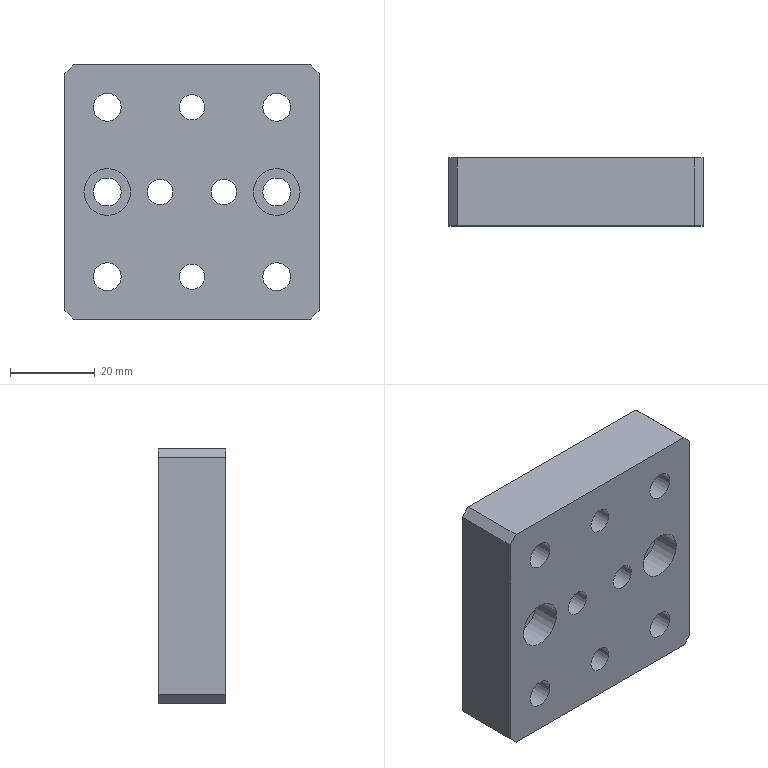Component | SolidWorks | UnitFixingPlate001-1 | 1 solid | 48 faces | box 60 x 16 x 60 mm | volume 49897 mm3 | cylinder 32 | plane 16 | commonest cylinder face diameters 11 x12 6.6 x12 6 x8 | material 6061 Alloy
build123d program:
from build123d import *

# Parameters (mm, degrees)
SKETCH1_W                                          = 60
SKETCH1_H                                          = 60
BOSS_EXTRUDE1_DEPTH                                = 8
HOLE_SIZE_ACCORDING_TO_TYPE_1_OF_HEXAG_D           = 6.6
HOLE_SIZE_ACCORDING_TO_TYPE_1_OF_HEXAG_CBORE_D     = 11
HOLE_SIZE_ACCORDING_TO_TYPE_1_OF_HEXAG_CBORE_DEPTH = 6.8
F_6_0_6_DIAMETER_HOLE1_D                           = 6
HOLE_SIZE_ACCORDING_TO_TYPE_2_HEXAGON_D            = 6.6
HOLE_SIZE_ACCORDING_TO_TYPE_2_HEXAGON_DEPTH        = 21
HOLE_SIZE_ACCORDING_TO_TYPE_2_HEXAGON_CBORE_D      = 11
HOLE_SIZE_ACCORDING_TO_TYPE_2_HEXAGON_CBORE_DEPTH  = 6.8
HOLE_SIZE_ACCORDING_TO_TYPE_2_HEXAGON_TIP          = 1.983
F_6_0_6_DIAMETER_HOLE2_D                           = 6
F_6_0_6_DIAMETER_HOLE2_DEPTH                       = 20
F_6_0_6_DIAMETER_HOLE2_TIP                         = 1.803
CHAMFER1_SIZE                                      = 2


with BuildPart() as part:
    # Sketch1 → Boss-Extrude1 (new, symmetric)
    with BuildSketch(Plane.XY):
        Rectangle(SKETCH1_W, SKETCH1_H)
    extrude(amount=BOSS_EXTRUDE1_DEPTH, both=True)

    # Hole Size _according to_ Type 1 of Hexag (through all)
    with Locations(Plane(origin=(0, 0, -8), x_dir=(-1, 0, 0), z_dir=(0, 0, -1))):
        with Locations((20, 0), (-20, 0)):
            CounterBoreHole(HOLE_SIZE_ACCORDING_TO_TYPE_1_OF_HEXAG_D / 2, HOLE_SIZE_ACCORDING_TO_TYPE_1_OF_HEXAG_CBORE_D / 2, HOLE_SIZE_ACCORDING_TO_TYPE_1_OF_HEXAG_CBORE_DEPTH)

    # 6.0 _6_ Diameter Hole1 (through all)
    with Locations(Plane(origin=(0, 0, -8), x_dir=(-1, 0, 0), z_dir=(0, 0, -1))):
        with Locations((-7.5, 0), (7.5, 0)):
            Hole(F_6_0_6_DIAMETER_HOLE1_D / 2)

    # Hole Size _ according to_ Type 2 Hexagon
    with Locations(Plane.XY.offset(8)):
        with Locations((-20, -20), (20, -20), (-20, 20), (20, 20)):
            CounterBoreHole(HOLE_SIZE_ACCORDING_TO_TYPE_2_HEXAGON_D / 2, HOLE_SIZE_ACCORDING_TO_TYPE_2_HEXAGON_CBORE_D / 2, HOLE_SIZE_ACCORDING_TO_TYPE_2_HEXAGON_CBORE_DEPTH, depth=HOLE_SIZE_ACCORDING_TO_TYPE_2_HEXAGON_DEPTH)
            with Locations((0, 0, -(HOLE_SIZE_ACCORDING_TO_TYPE_2_HEXAGON_DEPTH + HOLE_SIZE_ACCORDING_TO_TYPE_2_HEXAGON_TIP / 2))):  # 118° drill point
                Cone(0, HOLE_SIZE_ACCORDING_TO_TYPE_2_HEXAGON_D / 2, HOLE_SIZE_ACCORDING_TO_TYPE_2_HEXAGON_TIP, mode=Mode.SUBTRACT)

    # 6.0 _6_ Diameter Hole2
    with Locations(Plane.XY.offset(8)):
        with Locations((0, -20), (0, 20)):
            Hole(F_6_0_6_DIAMETER_HOLE2_D / 2, depth=F_6_0_6_DIAMETER_HOLE2_DEPTH)
            with Locations((0, 0, -(F_6_0_6_DIAMETER_HOLE2_DEPTH + F_6_0_6_DIAMETER_HOLE2_TIP / 2))):  # 118° drill point
                Cone(0, F_6_0_6_DIAMETER_HOLE2_D / 2, F_6_0_6_DIAMETER_HOLE2_TIP, mode=Mode.SUBTRACT)

    # Chamfer1
    chamfer1_edges = [part.edges().sort_by_distance(p)[0] for p in [
        (-30, 30, 0),
        (30, 30, 0),
        (30, -30, 0),
        (-30, -30, 0),
    ]]
    chamfer(chamfer1_edges, length=CHAMFER1_SIZE)


solid = part.part

# Placed as in the assembly
solid = solid.moved(Location((31.028, -68.899, 117.932), (-90, 0, 0)))